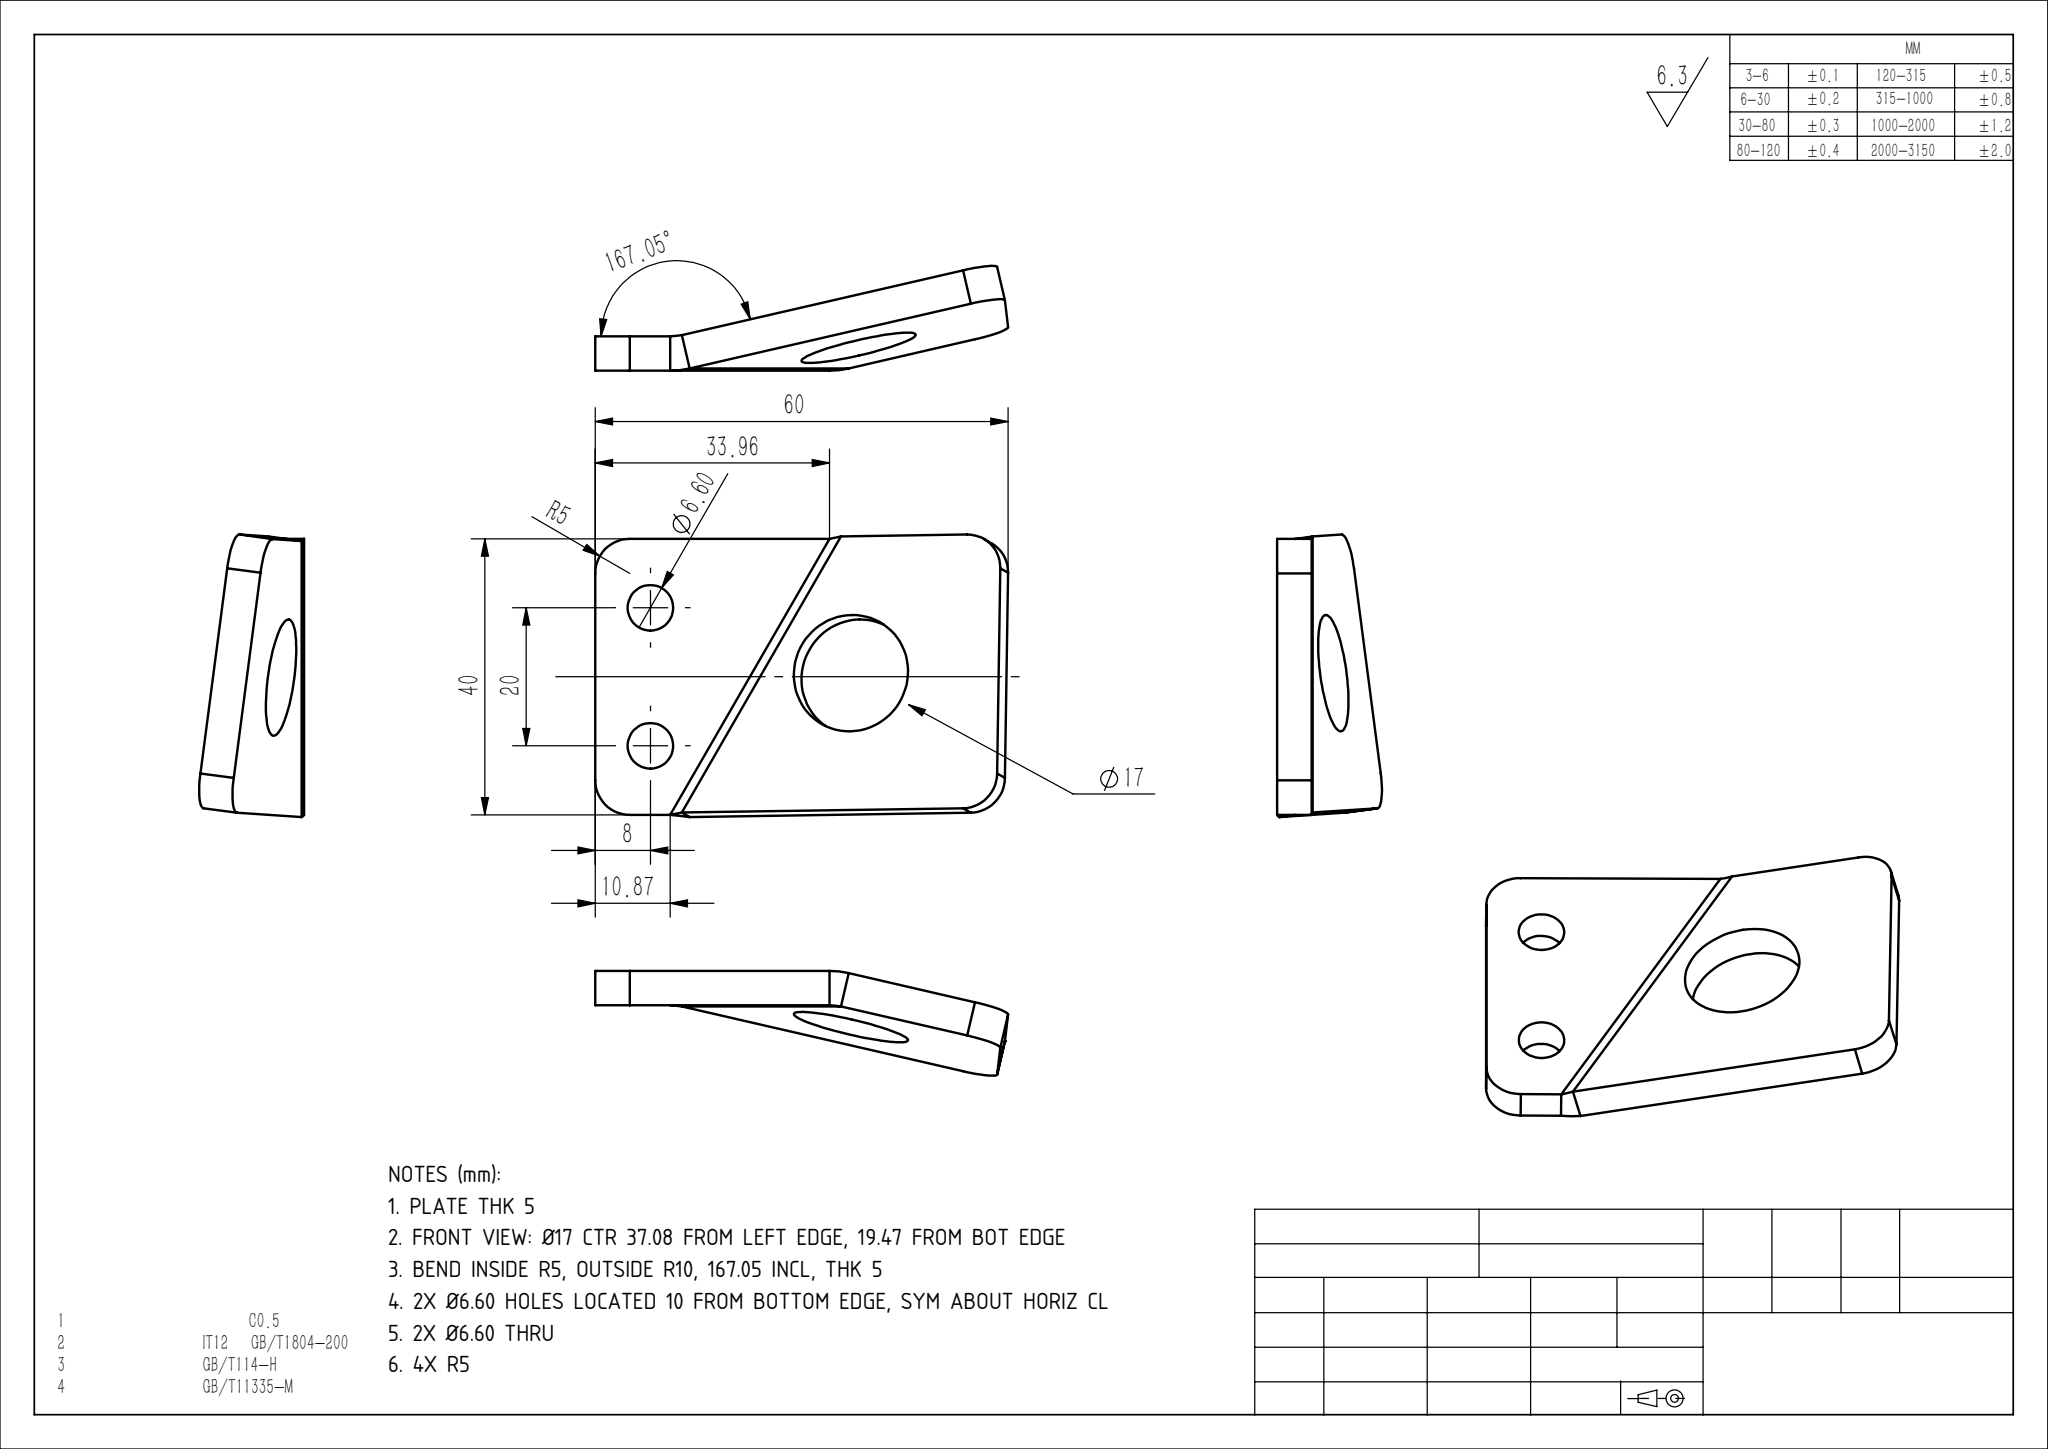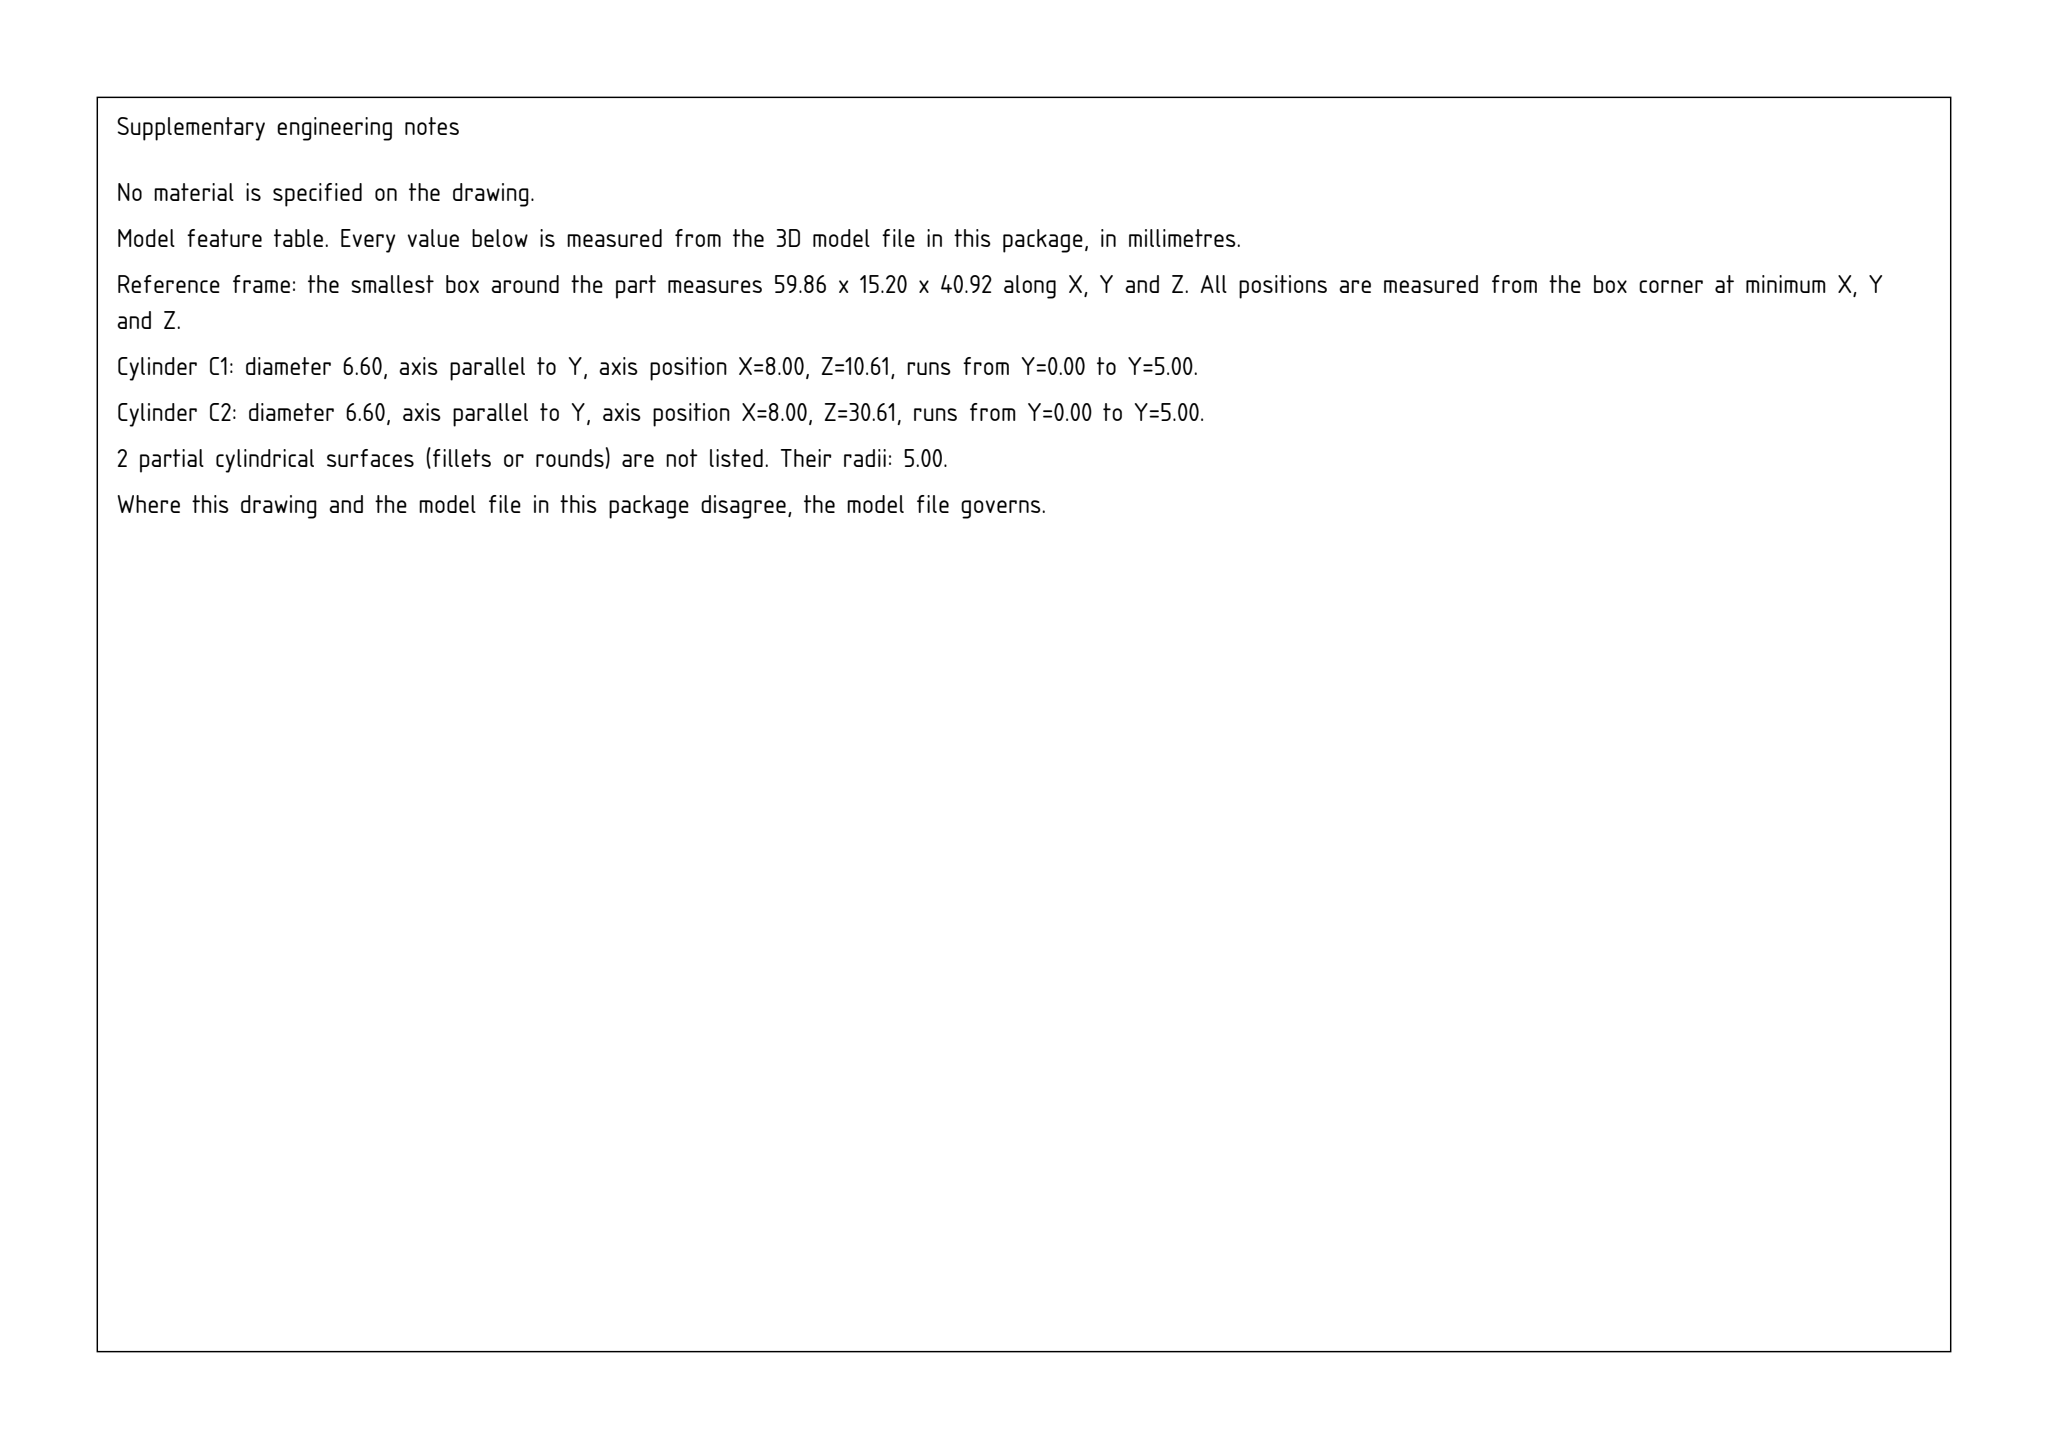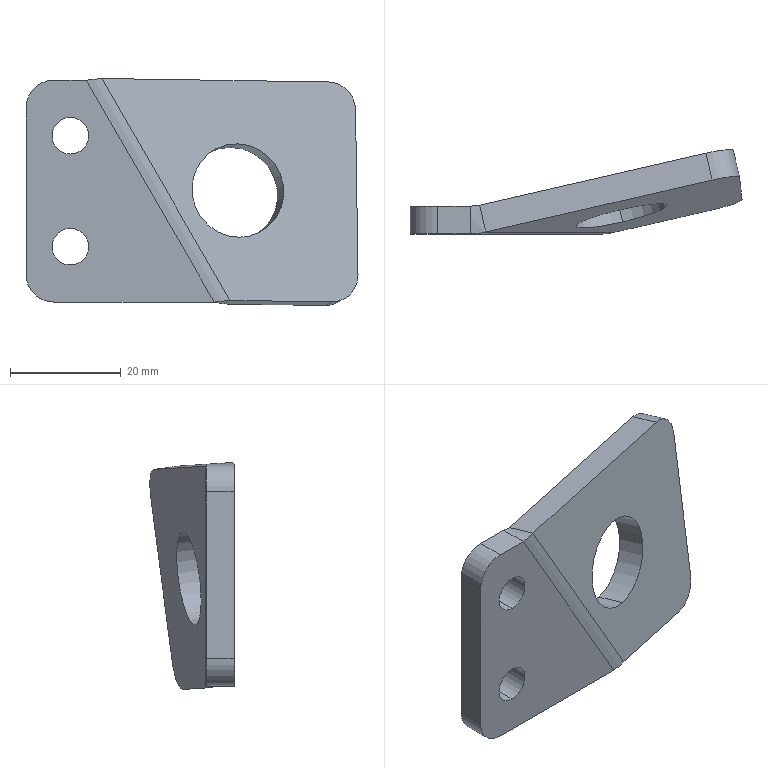Part | SolidWorks | mm | 1 solid | 24 faces | box 59.86 x 15.2 x 40.92 mm | volume 10416 mm3 | cylinder 12 | plane 10 | spline 2 | commonest cylinder face diameters 10 x5 6.6 x4 17 x2 20 x1
Drawing notes:
PLATE THK 5 | from the solid: Parallel faces at y=0 and y=5; all Ø6.60 holes 5 deep
FRONT VIEW: Ø17 CTR 37.08 FROM LEFT EDGE, 19.47 FROM BOT EDGE | from the solid: Ø17 cyl axis Y at x=37.08, z=20.45; part edges at x=0 and z=0.98 (40 wide to z=40.98)
BEND INSIDE R5, OUTSIDE R10, 167.05 INCL, THK 5 | from the solid: Coaxial cyls Ø10 (L=41.63) and Ø20 (L=42.28) about same axis at y=10, x=-1.4; faces y=0/y=5
2X Ø6.60 HOLES LOCATED 10 FROM BOTTOM EDGE, SYM ABOUT HORIZ CL | from the solid: Ø6.6 y-axis cyls at z=10.98 & 30.98; faces z=0.98 & 40.98 (40 wide) -> 10 & 30 from bottom edge, CL at 20.98
2X Ø6.60 THRU | from the solid: two Ø6.6 cylinders, axis y, length 5.0 = plate thk (planes y=0 and y=5)
4X R5 | from the solid: four Ø10 y-axis corner cyls at (5,5.98),(5,35.98),(53.42,35.07),(53.87,5.33)
STEP:
#1=CARTESIAN_POINT('',(8.,0.,6.7));
#2=VERTEX_POINT('',#1);
#3=CARTESIAN_POINT('',(8.,0.,13.3));
#4=VERTEX_POINT('',#3);
#5=CARTESIAN_POINT('',(8.,0.,10.));
#6=DIRECTION('',(0.,1.,0.));
#7=DIRECTION('',(0.,0.,1.));
#8=AXIS2_PLACEMENT_3D('',#5,#6,#7);
#9=CIRCLE('',#8,3.3);
#10=EDGE_CURVE('',#2,#4,#9,.T.);
#11=ORIENTED_EDGE('',*,*,#10,.F.);
#12=CARTESIAN_POINT('',(8.,5.,6.7));
#13=VERTEX_POINT('',#12);
#14=CARTESIAN_POINT('',(8.,5.,6.7));
#15=DIRECTION('',(0.,1.,0.));
#16=VECTOR('',#15,1000.);
#17=LINE('',#14,#16);
#18=EDGE_CURVE('',#2,#13,#17,.T.);
#19=ORIENTED_EDGE('',*,*,#18,.T.);
#20=CARTESIAN_POINT('',(8.,5.,13.3));
#21=VERTEX_POINT('',#20);
#22=CARTESIAN_POINT('',(8.,5.,10.));
#23=DIRECTION('',(0.,1.,0.));
#24=DIRECTION('',(0.,0.,1.));
#25=AXIS2_PLACEMENT_3D('',#22,#23,#24);
#26=CIRCLE('',#25,3.3);
#27=EDGE_CURVE('',#13,#21,#26,.T.);
#28=ORIENTED_EDGE('',*,*,#27,.T.);
#29=CARTESIAN_POINT('',(8.,5.,13.3));
#30=DIRECTION('',(0.,1.,0.));
#31=VECTOR('',#30,1000.);
#32=LINE('',#29,#31);
#33=EDGE_CURVE('',#4,#21,#32,.T.);
#34=ORIENTED_EDGE('',*,*,#33,.F.);
#35=EDGE_LOOP('',(#11,#19,#28,#34));
#36=FACE_OUTER_BOUND('',#35,.T.);
#37=CARTESIAN_POINT('',(8.,5.,10.));
#38=DIRECTION('',(0.,1.,0.));
#39=DIRECTION('',(0.,0.,1.));
#40=AXIS2_PLACEMENT_3D('',#37,#38,#39);
#41=CYLINDRICAL_SURFACE('',#40,3.3);
#42=ADVANCED_FACE('',(#36),#41,.F.);
#43=CARTESIAN_POINT('',(8.,0.,26.7));
#44=VERTEX_POINT('',#43);
#45=CARTESIAN_POINT('',(8.,0.,33.3));
#46=VERTEX_POINT('',#45);
#47=CARTESIAN_POINT('',(8.,0.,30.));
#48=DIRECTION('',(0.,1.,0.));
#49=DIRECTION('',(0.,0.,1.));
#50=AXIS2_PLACEMENT_3D('',#47,#48,#49);
#51=CIRCLE('',#50,3.3);
#52=EDGE_CURVE('',#44,#46,#51,.T.);
#53=ORIENTED_EDGE('',*,*,#52,.F.);
#54=CARTESIAN_POINT('',(8.,5.,26.7));
#55=VERTEX_POINT('',#54);
#56=CARTESIAN_POINT('',(8.,5.,26.7));
#57=DIRECTION('',(0.,1.,0.));
#58=VECTOR('',#57,1000.);
#59=LINE('',#56,#58);
#60=EDGE_CURVE('',#44,#55,#59,.T.);
#61=ORIENTED_EDGE('',*,*,#60,.T.);
#62=CARTESIAN_POINT('',(8.,5.,33.3));
#63=VERTEX_POINT('',#62);
#64=CARTESIAN_POINT('',(8.,5.,30.));
#65=DIRECTION('',(0.,1.,0.));
#66=DIRECTION('',(0.,0.,1.));
#67=AXIS2_PLACEMENT_3D('',#64,#65,#66);
#68=CIRCLE('',#67,3.3);
#69=EDGE_CURVE('',#55,#63,#68,.T.);
#70=ORIENTED_EDGE('',*,*,#69,.T.);
#71=CARTESIAN_POINT('',(8.,5.,33.3));
#72=DIRECTION('',(0.,1.,0.));
#73=VECTOR('',#72,1000.);
#74=LINE('',#71,#73);
#75=EDGE_CURVE('',#46,#63,#74,.T.);
#76=ORIENTED_EDGE('',*,*,#75,.F.);
#77=EDGE_LOOP('',(#53,#61,#70,#76));
#78=FACE_OUTER_BOUND('',#77,.T.);
#79=CARTESIAN_POINT('',(8.,5.,30.));
#80=DIRECTION('',(0.,1.,0.));
#81=DIRECTION('',(0.,0.,1.));
#82=AXIS2_PLACEMENT_3D('',#79,#80,#81);
#83=CYLINDRICAL_SURFACE('',#82,3.3);
#84=ADVANCED_FACE('',(#78),#83,.F.);
#85=CARTESIAN_POINT('',(36.954,9.256,27.896));
#86=VERTEX_POINT('',#85);
#87=CARTESIAN_POINT('',(37.205,7.056,11.041));
#88=VERTEX_POINT('',#87);
#89=CARTESIAN_POINT('',(37.08,8.156,19.469));
#90=DIRECTION('',(0.2241,-0.9659,0.1294));
#91=DIRECTION('',(0.01475,-0.1294,-0.9915));
#92=AXIS2_PLACEMENT_3D('',#89,#90,#91);
#93=CIRCLE('',#92,8.5);
#94=EDGE_CURVE('',#86,#88,#93,.T.);
#95=ORIENTED_EDGE('',*,*,#94,.F.);
#96=CARTESIAN_POINT('',(38.075,4.426,28.543));
#97=VERTEX_POINT('',#96);
#98=CARTESIAN_POINT('',(36.954,9.256,27.896));
#99=DIRECTION('',(0.2241,-0.9659,0.1294));
#100=VECTOR('',#99,1000.);
#101=LINE('',#98,#100);
#102=EDGE_CURVE('',#86,#97,#101,.T.);
#103=ORIENTED_EDGE('',*,*,#102,.T.);
#104=CARTESIAN_POINT('',(38.326,2.226,11.688));
#105=VERTEX_POINT('',#104);
#106=CARTESIAN_POINT('',(38.201,3.326,20.116));
#107=DIRECTION('',(0.2241,-0.9659,0.1294));
#108=DIRECTION('',(0.01475,-0.1294,-0.9915));
#109=AXIS2_PLACEMENT_3D('',#106,#107,#108);
#110=CIRCLE('',#109,8.5);
#111=EDGE_CURVE('',#97,#105,#110,.T.);
#112=ORIENTED_EDGE('',*,*,#111,.T.);
#113=CARTESIAN_POINT('',(37.205,7.056,11.041));
#114=DIRECTION('',(0.2241,-0.9659,0.1294));
#115=VECTOR('',#114,1000.);
#116=LINE('',#113,#115);
#117=EDGE_CURVE('',#88,#105,#116,.T.);
#118=ORIENTED_EDGE('',*,*,#117,.F.);
#119=EDGE_LOOP('',(#95,#103,#112,#118));
#120=FACE_OUTER_BOUND('',#119,.T.);
#121=CARTESIAN_POINT('',(37.08,8.156,19.469));
#122=DIRECTION('',(0.2241,-0.9659,0.1294));
#123=DIRECTION('',(0.01475,-0.1294,-0.9915));
#124=AXIS2_PLACEMENT_3D('',#121,#122,#123);
#125=CYLINDRICAL_SURFACE('',#124,8.5);
#126=ADVANCED_FACE('',(#120),#125,.F.);
#127=CARTESIAN_POINT('',(36.769,0.3407,0.3123));
#128=VERTEX_POINT('',#127);
#129=CARTESIAN_POINT('',(55.061,4.548,0.03537));
#130=VERTEX_POINT('',#129);
#131=CARTESIAN_POINT('',(1.467,-7.779,0.8469));
#132=DIRECTION('',(0.9744,0.2241,-0.01475));
#133=VECTOR('',#132,1000.);
#134=LINE('',#131,#133);
#135=EDGE_CURVE('',#128,#130,#134,.T.);
#136=ORIENTED_EDGE('',*,*,#135,.F.);
#137=CARTESIAN_POINT('',(35.648,5.17,-0.3347));
#138=VERTEX_POINT('',#137);
#139=CARTESIAN_POINT('',(36.769,0.3407,0.3123));
#140=CARTESIAN_POINT('',(36.395,1.951,0.09666));
#141=CARTESIAN_POINT('',(36.021,3.56,-0.119));
#142=CARTESIAN_POINT('',(35.648,5.17,-0.3347));
#143=B_SPLINE_CURVE_WITH_KNOTS('',3,(#139,#140,#141,#142),.UNSPECIFIED.,.F.,.F.,(4,4),(0.,1.),.UNSPECIFIED.);
#144=EDGE_CURVE('',#128,#138,#143,.T.);
#145=ORIENTED_EDGE('',*,*,#144,.T.);
#146=CARTESIAN_POINT('',(53.941,9.378,-0.6117));
#147=VERTEX_POINT('',#146);
#148=CARTESIAN_POINT('',(0.3461,-2.95,0.1998));
#149=DIRECTION('',(0.9744,0.2241,-0.01475));
#150=VECTOR('',#149,1000.);
#151=LINE('',#148,#150);
#152=EDGE_CURVE('',#138,#147,#151,.T.);
#153=ORIENTED_EDGE('',*,*,#152,.T.);
#154=CARTESIAN_POINT('',(53.941,9.378,-0.6117));
#155=DIRECTION('',(-0.2241,0.9659,-0.1294));
#156=VECTOR('',#155,1000.);
#157=LINE('',#154,#156);
#158=EDGE_CURVE('',#130,#147,#157,.T.);
#159=ORIENTED_EDGE('',*,*,#158,.F.);
#160=EDGE_LOOP('',(#136,#145,#153,#159));
#161=FACE_OUTER_BOUND('',#160,.T.);
#162=CARTESIAN_POINT('',(0.3461,-2.95,0.1998));
#163=DIRECTION('',(-0.01475,0.1294,0.9915));
#164=DIRECTION('',(0.9744,0.2241,-0.01475));
#165=AXIS2_PLACEMENT_3D('',#162,#163,#164);
#166=PLANE('',#165);
#167=ADVANCED_FACE('',(#161),#166,.F.);
#168=CARTESIAN_POINT('',(12.554,5.17,39.665));
#169=VERTEX_POINT('',#168);
#170=CARTESIAN_POINT('',(53.35,14.554,39.048));
#171=VERTEX_POINT('',#170);
#172=CARTESIAN_POINT('',(-0.2441,2.227,39.859));
#173=DIRECTION('',(0.9744,0.2241,-0.01475));
#174=VECTOR('',#173,1000.);
#175=LINE('',#172,#174);
#176=EDGE_CURVE('',#169,#171,#175,.T.);
#177=ORIENTED_EDGE('',*,*,#176,.F.);
#178=CARTESIAN_POINT('',(13.675,0.3407,40.312));
#179=VERTEX_POINT('',#178);
#180=CARTESIAN_POINT('',(12.554,5.17,39.665));
#181=CARTESIAN_POINT('',(12.927,3.56,39.881));
#182=CARTESIAN_POINT('',(13.301,1.951,40.097));
#183=CARTESIAN_POINT('',(13.675,0.3407,40.312));
#184=B_SPLINE_CURVE_WITH_KNOTS('',3,(#180,#181,#182,#183),.UNSPECIFIED.,.F.,.F.,(4,4),(0.,1.),.UNSPECIFIED.);
#185=EDGE_CURVE('',#169,#179,#184,.T.);
#186=ORIENTED_EDGE('',*,*,#185,.T.);
#187=CARTESIAN_POINT('',(54.471,9.725,39.695));
#188=VERTEX_POINT('',#187);
#189=CARTESIAN_POINT('',(0.8766,-2.603,40.506));
#190=DIRECTION('',(0.9744,0.2241,-0.01475));
#191=VECTOR('',#190,1000.);
#192=LINE('',#189,#191);
#193=EDGE_CURVE('',#179,#188,#192,.T.);
#194=ORIENTED_EDGE('',*,*,#193,.T.);
#195=CARTESIAN_POINT('',(53.35,14.554,39.048));
#196=DIRECTION('',(-0.2241,0.9659,-0.1294));
#197=VECTOR('',#196,1000.);
#198=LINE('',#195,#197);
#199=EDGE_CURVE('',#188,#171,#198,.T.);
#200=ORIENTED_EDGE('',*,*,#199,.T.);
#201=EDGE_LOOP('',(#177,#186,#194,#200));
#202=FACE_OUTER_BOUND('',#201,.T.);
#203=CARTESIAN_POINT('',(-0.2441,2.227,39.859));
#204=DIRECTION('',(-0.01475,0.1294,0.9915));
#205=DIRECTION('',(0.9744,0.2241,-0.01475));
#206=AXIS2_PLACEMENT_3D('',#203,#204,#205);
#207=PLANE('',#206);
#208=ADVANCED_FACE('',(#202),#207,.T.);
#209=CARTESIAN_POINT('',(37.08,8.156,19.469));
#210=DIRECTION('',(0.2241,-0.9659,0.1294));
#211=DIRECTION('',(0.01475,-0.1294,-0.9915));
#212=AXIS2_PLACEMENT_3D('',#209,#210,#211);
#213=CIRCLE('',#212,8.5);
#214=EDGE_CURVE('',#88,#86,#213,.T.);
#215=ORIENTED_EDGE('',*,*,#214,.T.);
#216=ORIENTED_EDGE('',*,*,#94,.T.);
#217=EDGE_LOOP('',(#215,#216));
#218=FACE_BOUND('',#217,.T.);
#219=ORIENTED_EDGE('',*,*,#152,.F.);
#220=CARTESIAN_POINT('',(9.271,5.17,45.352));
#221=DIRECTION('',(-0.5,0.,0.866));
#222=VECTOR('',#221,1000.);
#223=LINE('',#220,#222);
#224=EDGE_CURVE('',#138,#169,#223,.T.);
#225=ORIENTED_EDGE('',*,*,#224,.T.);
#226=ORIENTED_EDGE('',*,*,#176,.T.);
#227=CARTESIAN_POINT('',(58.296,15.028,34.016));
#228=VERTEX_POINT('',#227);
#229=CARTESIAN_POINT('',(53.424,13.907,34.09));
#230=DIRECTION('',(-0.2241,0.9659,-0.1294));
#231=DIRECTION('',(-0.01475,0.1294,0.9915));
#232=AXIS2_PLACEMENT_3D('',#229,#230,#231);
#233=CIRCLE('',#232,5.);
#234=EDGE_CURVE('',#171,#228,#233,.T.);
#235=ORIENTED_EDGE('',*,*,#234,.T.);
#236=CARTESIAN_POINT('',(58.739,11.146,4.272));
#237=VERTEX_POINT('',#236);
#238=CARTESIAN_POINT('',(58.223,15.675,38.974));
#239=DIRECTION('',(0.01475,-0.1294,-0.9915));
#240=VECTOR('',#239,1000.);
#241=LINE('',#238,#240);
#242=EDGE_CURVE('',#228,#237,#241,.T.);
#243=ORIENTED_EDGE('',*,*,#242,.T.);
#244=CARTESIAN_POINT('',(53.867,10.025,4.346));
#245=DIRECTION('',(-0.2241,0.9659,-0.1294));
#246=DIRECTION('',(-0.01475,0.1294,0.9915));
#247=AXIS2_PLACEMENT_3D('',#244,#245,#246);
#248=CIRCLE('',#247,5.);
#249=EDGE_CURVE('',#237,#147,#248,.T.);
#250=ORIENTED_EDGE('',*,*,#249,.T.);
#251=EDGE_LOOP('',(#219,#225,#226,#235,#243,#250));
#252=FACE_OUTER_BOUND('',#251,.T.);
#253=CARTESIAN_POINT('',(-0.2441,2.227,39.859));
#254=DIRECTION('',(-0.2241,0.9659,-0.1294));
#255=DIRECTION('',(-0.01475,0.1294,0.9915));
#256=AXIS2_PLACEMENT_3D('',#253,#254,#255);
#257=PLANE('',#256);
#258=ADVANCED_FACE('',(#218,#252),#257,.T.);
#259=ORIENTED_EDGE('',*,*,#199,.F.);
#260=CARTESIAN_POINT('',(59.417,10.199,34.663));
#261=VERTEX_POINT('',#260);
#262=CARTESIAN_POINT('',(54.545,9.078,34.737));
#263=DIRECTION('',(-0.2241,0.9659,-0.1294));
#264=DIRECTION('',(-0.01475,0.1294,0.9915));
#265=AXIS2_PLACEMENT_3D('',#262,#263,#264);
#266=CIRCLE('',#265,5.);
#267=EDGE_CURVE('',#188,#261,#266,.T.);
#268=ORIENTED_EDGE('',*,*,#267,.T.);
#269=CARTESIAN_POINT('',(58.296,15.028,34.016));
#270=DIRECTION('',(-0.2241,0.9659,-0.1294));
#271=VECTOR('',#270,1000.);
#272=LINE('',#269,#271);
#273=EDGE_CURVE('',#261,#228,#272,.T.);
#274=ORIENTED_EDGE('',*,*,#273,.T.);
#275=ORIENTED_EDGE('',*,*,#234,.F.);
#276=EDGE_LOOP('',(#259,#268,#274,#275));
#277=FACE_OUTER_BOUND('',#276,.T.);
#278=CARTESIAN_POINT('',(53.424,13.907,34.09));
#279=DIRECTION('',(-0.2241,0.9659,-0.1294));
#280=DIRECTION('',(-0.01475,0.1294,0.9915));
#281=AXIS2_PLACEMENT_3D('',#278,#279,#280);
#282=CYLINDRICAL_SURFACE('',#281,5.);
#283=ADVANCED_FACE('',(#277),#282,.T.);
#284=ORIENTED_EDGE('',*,*,#273,.F.);
#285=CARTESIAN_POINT('',(59.86,6.316,4.919));
#286=VERTEX_POINT('',#285);
#287=CARTESIAN_POINT('',(59.343,10.846,39.621));
#288=DIRECTION('',(0.01475,-0.1294,-0.9915));
#289=VECTOR('',#288,1000.);
#290=LINE('',#287,#289);
#291=EDGE_CURVE('',#261,#286,#290,.T.);
#292=ORIENTED_EDGE('',*,*,#291,.T.);
#293=CARTESIAN_POINT('',(58.739,11.146,4.272));
#294=DIRECTION('',(-0.2241,0.9659,-0.1294));
#295=VECTOR('',#294,1000.);
#296=LINE('',#293,#295);
#297=EDGE_CURVE('',#286,#237,#296,.T.);
#298=ORIENTED_EDGE('',*,*,#297,.T.);
#299=ORIENTED_EDGE('',*,*,#242,.F.);
#300=EDGE_LOOP('',(#284,#292,#298,#299));
#301=FACE_OUTER_BOUND('',#300,.T.);
#302=CARTESIAN_POINT('',(58.223,15.675,38.974));
#303=DIRECTION('',(0.9744,0.2241,-0.01475));
#304=DIRECTION('',(0.01475,-0.1294,-0.9915));
#305=AXIS2_PLACEMENT_3D('',#302,#303,#304);
#306=PLANE('',#305);
#307=ADVANCED_FACE('',(#301),#306,.T.);
#308=ORIENTED_EDGE('',*,*,#102,.F.);
#309=ORIENTED_EDGE('',*,*,#214,.F.);
#310=ORIENTED_EDGE('',*,*,#117,.T.);
#311=CARTESIAN_POINT('',(38.201,3.326,20.116));
#312=DIRECTION('',(0.2241,-0.9659,0.1294));
#313=DIRECTION('',(0.01475,-0.1294,-0.9915));
#314=AXIS2_PLACEMENT_3D('',#311,#312,#313);
#315=CIRCLE('',#314,8.5);
#316=EDGE_CURVE('',#105,#97,#315,.T.);
#317=ORIENTED_EDGE('',*,*,#316,.T.);
#318=EDGE_LOOP('',(#308,#309,#310,#317));
#319=FACE_OUTER_BOUND('',#318,.T.);
#320=CARTESIAN_POINT('',(37.08,8.156,19.469));
#321=DIRECTION('',(0.2241,-0.9659,0.1294));
#322=DIRECTION('',(0.01475,-0.1294,-0.9915));
#323=AXIS2_PLACEMENT_3D('',#320,#321,#322);
#324=CYLINDRICAL_SURFACE('',#323,8.5);
#325=ADVANCED_FACE('',(#319),#324,.F.);
#326=CARTESIAN_POINT('',(54.987,5.195,4.993));
#327=DIRECTION('',(-0.2241,0.9659,-0.1294));
#328=DIRECTION('',(-0.01475,0.1294,0.9915));
#329=AXIS2_PLACEMENT_3D('',#326,#327,#328);
#330=CIRCLE('',#329,5.);
#331=EDGE_CURVE('',#286,#130,#330,.T.);
#332=ORIENTED_EDGE('',*,*,#331,.T.);
#333=ORIENTED_EDGE('',*,*,#158,.T.);
#334=ORIENTED_EDGE('',*,*,#249,.F.);
#335=ORIENTED_EDGE('',*,*,#297,.F.);
#336=EDGE_LOOP('',(#332,#333,#334,#335));
#337=FACE_OUTER_BOUND('',#336,.T.);
#338=CARTESIAN_POINT('',(53.867,10.025,4.346));
#339=DIRECTION('',(-0.2241,0.9659,-0.1294));
#340=DIRECTION('',(-0.01475,0.1294,0.9915));
#341=AXIS2_PLACEMENT_3D('',#338,#339,#340);
#342=CYLINDRICAL_SURFACE('',#341,5.);
#343=ADVANCED_FACE('',(#337),#342,.T.);
#344=CARTESIAN_POINT('',(10.391,0.3407,45.999));
#345=DIRECTION('',(-0.5,0.,0.866));
#346=VECTOR('',#345,1000.);
#347=LINE('',#344,#346);
#348=EDGE_CURVE('',#128,#179,#347,.T.);
#349=ORIENTED_EDGE('',*,*,#348,.F.);
#350=ORIENTED_EDGE('',*,*,#135,.T.);
#351=ORIENTED_EDGE('',*,*,#331,.F.);
#352=ORIENTED_EDGE('',*,*,#291,.F.);
#353=ORIENTED_EDGE('',*,*,#267,.F.);
#354=ORIENTED_EDGE('',*,*,#193,.F.);
#355=EDGE_LOOP('',(#349,#350,#351,#352,#353,#354));
#356=FACE_OUTER_BOUND('',#355,.T.);
#357=ORIENTED_EDGE('',*,*,#316,.F.);
#358=ORIENTED_EDGE('',*,*,#111,.F.);
#359=EDGE_LOOP('',(#357,#358));
#360=FACE_BOUND('',#359,.T.);
#361=CARTESIAN_POINT('',(0.8766,-2.603,40.506));
#362=DIRECTION('',(-0.2241,0.9659,-0.1294));
#363=DIRECTION('',(-0.01475,0.1294,0.9915));
#364=AXIS2_PLACEMENT_3D('',#361,#362,#363);
#365=PLANE('',#364);
#366=ADVANCED_FACE('',(#356,#360),#365,.F.);
#367=ORIENTED_EDGE('',*,*,#60,.F.);
#368=CARTESIAN_POINT('',(8.,0.,30.));
#369=DIRECTION('',(0.,1.,0.));
#370=DIRECTION('',(0.,0.,1.));
#371=AXIS2_PLACEMENT_3D('',#368,#369,#370);
#372=CIRCLE('',#371,3.3);
#373=EDGE_CURVE('',#46,#44,#372,.T.);
#374=ORIENTED_EDGE('',*,*,#373,.F.);
#375=ORIENTED_EDGE('',*,*,#75,.T.);
#376=CARTESIAN_POINT('',(8.,5.,30.));
#377=DIRECTION('',(0.,1.,0.));
#378=DIRECTION('',(0.,0.,1.));
#379=AXIS2_PLACEMENT_3D('',#376,#377,#378);
#380=CIRCLE('',#379,3.3);
#381=EDGE_CURVE('',#63,#55,#380,.T.);
#382=ORIENTED_EDGE('',*,*,#381,.T.);
#383=EDGE_LOOP('',(#367,#374,#375,#382));
#384=FACE_OUTER_BOUND('',#383,.T.);
#385=CARTESIAN_POINT('',(8.,5.,30.));
#386=DIRECTION('',(0.,1.,0.));
#387=DIRECTION('',(0.,0.,1.));
#388=AXIS2_PLACEMENT_3D('',#385,#386,#387);
#389=CYLINDRICAL_SURFACE('',#388,3.3);
#390=ADVANCED_FACE('',(#384),#389,.F.);
#391=ORIENTED_EDGE('',*,*,#18,.F.);
#392=CARTESIAN_POINT('',(8.,0.,10.));
#393=DIRECTION('',(0.,1.,0.));
#394=DIRECTION('',(0.,0.,1.));
#395=AXIS2_PLACEMENT_3D('',#392,#393,#394);
#396=CIRCLE('',#395,3.3);
#397=EDGE_CURVE('',#4,#2,#396,.T.);
#398=ORIENTED_EDGE('',*,*,#397,.F.);
#399=ORIENTED_EDGE('',*,*,#33,.T.);
#400=CARTESIAN_POINT('',(8.,5.,10.));
#401=DIRECTION('',(0.,1.,0.));
#402=DIRECTION('',(0.,0.,1.));
#403=AXIS2_PLACEMENT_3D('',#400,#401,#402);
#404=CIRCLE('',#403,3.3);
#405=EDGE_CURVE('',#21,#13,#404,.T.);
#406=ORIENTED_EDGE('',*,*,#405,.T.);
#407=EDGE_LOOP('',(#391,#398,#399,#406));
#408=FACE_OUTER_BOUND('',#407,.T.);
#409=CARTESIAN_POINT('',(8.,5.,10.));
#410=DIRECTION('',(0.,1.,0.));
#411=DIRECTION('',(0.,0.,1.));
#412=AXIS2_PLACEMENT_3D('',#409,#410,#411);
#413=CYLINDRICAL_SURFACE('',#412,3.3);
#414=ADVANCED_FACE('',(#408),#413,.F.);
#415=CARTESIAN_POINT('',(0.,0.,35.));
#416=VERTEX_POINT('',#415);
#417=CARTESIAN_POINT('',(0.,5.,35.));
#418=VERTEX_POINT('',#417);
#419=CARTESIAN_POINT('',(0.,5.,35.));
#420=DIRECTION('',(0.,1.,0.));
#421=VECTOR('',#420,1000.);
#422=LINE('',#419,#421);
#423=EDGE_CURVE('',#416,#418,#422,.T.);
#424=ORIENTED_EDGE('',*,*,#423,.F.);
#425=CARTESIAN_POINT('',(5.,0.,40.));
#426=VERTEX_POINT('',#425);
#427=CARTESIAN_POINT('',(5.,0.,35.));
#428=DIRECTION('',(0.,1.,0.));
#429=DIRECTION('',(0.,0.,1.));
#430=AXIS2_PLACEMENT_3D('',#427,#428,#429);
#431=CIRCLE('',#430,5.);
#432=EDGE_CURVE('',#416,#426,#431,.T.);
#433=ORIENTED_EDGE('',*,*,#432,.T.);
#434=CARTESIAN_POINT('',(5.,5.,40.));
#435=VERTEX_POINT('',#434);
#436=CARTESIAN_POINT('',(5.,5.,40.));
#437=DIRECTION('',(0.,1.,0.));
#438=VECTOR('',#437,1000.);
#439=LINE('',#436,#438);
#440=EDGE_CURVE('',#426,#435,#439,.T.);
#441=ORIENTED_EDGE('',*,*,#440,.T.);
#442=CARTESIAN_POINT('',(5.,5.,35.));
#443=DIRECTION('',(0.,1.,0.));
#444=DIRECTION('',(0.,0.,1.));
#445=AXIS2_PLACEMENT_3D('',#442,#443,#444);
#446=CIRCLE('',#445,5.);
#447=EDGE_CURVE('',#418,#435,#446,.T.);
#448=ORIENTED_EDGE('',*,*,#447,.F.);
#449=EDGE_LOOP('',(#424,#433,#441,#448));
#450=FACE_OUTER_BOUND('',#449,.T.);
#451=CARTESIAN_POINT('',(5.,5.,35.));
#452=DIRECTION('',(0.,1.,0.));
#453=DIRECTION('',(0.,0.,1.));
#454=AXIS2_PLACEMENT_3D('',#451,#452,#453);
#455=CYLINDRICAL_SURFACE('',#454,5.);
#456=ADVANCED_FACE('',(#450),#455,.T.);
#457=CARTESIAN_POINT('',(0.,0.,5.));
#458=VERTEX_POINT('',#457);
#459=CARTESIAN_POINT('',(0.,5.,5.));
#460=VERTEX_POINT('',#459);
#461=CARTESIAN_POINT('',(0.,5.,5.));
#462=DIRECTION('',(0.,1.,0.));
#463=VECTOR('',#462,1000.);
#464=LINE('',#461,#463);
#465=EDGE_CURVE('',#458,#460,#464,.T.);
#466=ORIENTED_EDGE('',*,*,#465,.F.);
#467=CARTESIAN_POINT('',(0.,0.,40.));
#468=DIRECTION('',(0.,0.,-1.));
#469=VECTOR('',#468,1000.);
#470=LINE('',#467,#469);
#471=EDGE_CURVE('',#416,#458,#470,.T.);
#472=ORIENTED_EDGE('',*,*,#471,.F.);
#473=ORIENTED_EDGE('',*,*,#423,.T.);
#474=CARTESIAN_POINT('',(0.,5.,40.));
#475=DIRECTION('',(0.,0.,-1.));
#476=VECTOR('',#475,1000.);
#477=LINE('',#474,#476);
#478=EDGE_CURVE('',#418,#460,#477,.T.);
#479=ORIENTED_EDGE('',*,*,#478,.T.);
#480=EDGE_LOOP('',(#466,#472,#473,#479));
#481=FACE_OUTER_BOUND('',#480,.T.);
#482=CARTESIAN_POINT('',(0.,5.,40.));
#483=DIRECTION('',(1.,0.,0.));
#484=DIRECTION('',(0.,0.,-1.));
#485=AXIS2_PLACEMENT_3D('',#482,#483,#484);
#486=PLANE('',#485);
#487=ADVANCED_FACE('',(#481),#486,.F.);
#488=CARTESIAN_POINT('',(5.,0.,0.));
#489=VERTEX_POINT('',#488);
#490=CARTESIAN_POINT('',(5.,5.,0.));
#491=VERTEX_POINT('',#490);
#492=CARTESIAN_POINT('',(5.,5.,0.));
#493=DIRECTION('',(0.,1.,0.));
#494=VECTOR('',#493,1000.);
#495=LINE('',#492,#494);
#496=EDGE_CURVE('',#489,#491,#495,.T.);
#497=ORIENTED_EDGE('',*,*,#496,.F.);
#498=CARTESIAN_POINT('',(5.,0.,5.));
#499=DIRECTION('',(0.,1.,0.));
#500=DIRECTION('',(0.,0.,1.));
#501=AXIS2_PLACEMENT_3D('',#498,#499,#500);
#502=CIRCLE('',#501,5.);
#503=EDGE_CURVE('',#489,#458,#502,.T.);
#504=ORIENTED_EDGE('',*,*,#503,.T.);
#505=ORIENTED_EDGE('',*,*,#465,.T.);
#506=CARTESIAN_POINT('',(5.,5.,5.));
#507=DIRECTION('',(0.,1.,0.));
#508=DIRECTION('',(0.,0.,1.));
#509=AXIS2_PLACEMENT_3D('',#506,#507,#508);
#510=CIRCLE('',#509,5.);
#511=EDGE_CURVE('',#491,#460,#510,.T.);
#512=ORIENTED_EDGE('',*,*,#511,.F.);
#513=EDGE_LOOP('',(#497,#504,#505,#512));
#514=FACE_OUTER_BOUND('',#513,.T.);
#515=CARTESIAN_POINT('',(5.,5.,5.));
#516=DIRECTION('',(0.,1.,0.));
#517=DIRECTION('',(0.,0.,1.));
#518=AXIS2_PLACEMENT_3D('',#515,#516,#517);
#519=CYLINDRICAL_SURFACE('',#518,5.);
#520=ADVANCED_FACE('',(#514),#519,.T.);
#521=CARTESIAN_POINT('',(33.96,5.,-0.));
#522=VERTEX_POINT('',#521);
#523=CARTESIAN_POINT('',(10.866,5.,40.));
#524=VERTEX_POINT('',#523);
#525=CARTESIAN_POINT('',(8.15,5.,44.705));
#526=DIRECTION('',(-0.5,0.,0.866));
#527=VECTOR('',#526,1000.);
#528=LINE('',#525,#527);
#529=EDGE_CURVE('',#522,#524,#528,.T.);
#530=ORIENTED_EDGE('',*,*,#529,.F.);
#531=CARTESIAN_POINT('',(0.,5.,0.));
#532=DIRECTION('',(1.,0.,0.));
#533=VECTOR('',#532,1000.);
#534=LINE('',#531,#533);
#535=EDGE_CURVE('',#491,#522,#534,.T.);
#536=ORIENTED_EDGE('',*,*,#535,.F.);
#537=ORIENTED_EDGE('',*,*,#511,.T.);
#538=ORIENTED_EDGE('',*,*,#478,.F.);
#539=ORIENTED_EDGE('',*,*,#447,.T.);
#540=CARTESIAN_POINT('',(0.,5.,40.));
#541=DIRECTION('',(1.,0.,0.));
#542=VECTOR('',#541,1000.);
#543=LINE('',#540,#542);
#544=EDGE_CURVE('',#435,#524,#543,.T.);
#545=ORIENTED_EDGE('',*,*,#544,.T.);
#546=EDGE_LOOP('',(#530,#536,#537,#538,#539,#545));
#547=FACE_OUTER_BOUND('',#546,.T.);
#548=ORIENTED_EDGE('',*,*,#405,.F.);
#549=ORIENTED_EDGE('',*,*,#27,.F.);
#550=EDGE_LOOP('',(#548,#549));
#551=FACE_BOUND('',#550,.T.);
#552=ORIENTED_EDGE('',*,*,#381,.F.);
#553=ORIENTED_EDGE('',*,*,#69,.F.);
#554=EDGE_LOOP('',(#552,#553));
#555=FACE_BOUND('',#554,.T.);
#556=CARTESIAN_POINT('',(0.,5.,40.));
#557=DIRECTION('',(0.,1.,0.));
#558=DIRECTION('',(0.,0.,1.));
#559=AXIS2_PLACEMENT_3D('',#556,#557,#558);
#560=PLANE('',#559);
#561=ADVANCED_FACE('',(#547,#551,#555),#560,.T.);
#562=CARTESIAN_POINT('',(33.96,0.,-0.));
#563=VERTEX_POINT('',#562);
#564=CARTESIAN_POINT('',(33.96,0.,-0.));
#565=CARTESIAN_POINT('',(33.96,5.,-0.));
#566=B_SPLINE_CURVE_WITH_KNOTS('',1,(#564,#565),.UNSPECIFIED.,.F.,.F.,(2,2),(0.,1.),.UNSPECIFIED.);
#567=EDGE_CURVE('',#563,#522,#566,.T.);
#568=ORIENTED_EDGE('',*,*,#567,.F.);
#569=CARTESIAN_POINT('',(0.,0.,0.));
#570=DIRECTION('',(1.,0.,0.));
#571=VECTOR('',#570,1000.);
#572=LINE('',#569,#571);
#573=EDGE_CURVE('',#489,#563,#572,.T.);
#574=ORIENTED_EDGE('',*,*,#573,.F.);
#575=ORIENTED_EDGE('',*,*,#496,.T.);
#576=ORIENTED_EDGE('',*,*,#535,.T.);
#577=EDGE_LOOP('',(#568,#574,#575,#576));
#578=FACE_OUTER_BOUND('',#577,.T.);
#579=CARTESIAN_POINT('',(0.,5.,0.));
#580=DIRECTION('',(0.,0.,1.));
#581=DIRECTION('',(1.,0.,0.));
#582=AXIS2_PLACEMENT_3D('',#579,#580,#581);
#583=PLANE('',#582);
#584=ADVANCED_FACE('',(#578),#583,.F.);
#585=ORIENTED_EDGE('',*,*,#373,.T.);
#586=ORIENTED_EDGE('',*,*,#52,.T.);
#587=EDGE_LOOP('',(#585,#586));
#588=FACE_BOUND('',#587,.T.);
#589=ORIENTED_EDGE('',*,*,#397,.T.);
#590=ORIENTED_EDGE('',*,*,#10,.T.);
#591=EDGE_LOOP('',(#589,#590));
#592=FACE_BOUND('',#591,.T.);
#593=ORIENTED_EDGE('',*,*,#573,.T.);
#594=CARTESIAN_POINT('',(10.866,0.,40.));
#595=VERTEX_POINT('',#594);
#596=CARTESIAN_POINT('',(8.15,0.,44.705));
#597=DIRECTION('',(-0.5,0.,0.866));
#598=VECTOR('',#597,1000.);
#599=LINE('',#596,#598);
#600=EDGE_CURVE('',#563,#595,#599,.T.);
#601=ORIENTED_EDGE('',*,*,#600,.T.);
#602=CARTESIAN_POINT('',(0.,0.,40.));
#603=DIRECTION('',(1.,0.,0.));
#604=VECTOR('',#603,1000.);
#605=LINE('',#602,#604);
#606=EDGE_CURVE('',#426,#595,#605,.T.);
#607=ORIENTED_EDGE('',*,*,#606,.F.);
#608=ORIENTED_EDGE('',*,*,#432,.F.);
#609=ORIENTED_EDGE('',*,*,#471,.T.);
#610=ORIENTED_EDGE('',*,*,#503,.F.);
#611=EDGE_LOOP('',(#593,#601,#607,#608,#609,#610));
#612=FACE_OUTER_BOUND('',#611,.T.);
#613=CARTESIAN_POINT('',(0.,0.,40.));
#614=DIRECTION('',(0.,1.,0.));
#615=DIRECTION('',(0.,0.,1.));
#616=AXIS2_PLACEMENT_3D('',#613,#614,#615);
#617=PLANE('',#616);
#618=ADVANCED_FACE('',(#588,#592,#612),#617,.F.);
#619=CARTESIAN_POINT('',(10.866,5.,40.));
#620=CARTESIAN_POINT('',(10.866,0.,40.));
#621=B_SPLINE_CURVE_WITH_KNOTS('',1,(#619,#620),.UNSPECIFIED.,.F.,.F.,(2,2),(0.,1.),.UNSPECIFIED.);
#622=EDGE_CURVE('',#524,#595,#621,.T.);
#623=ORIENTED_EDGE('',*,*,#622,.F.);
#624=ORIENTED_EDGE('',*,*,#544,.F.);
#625=ORIENTED_EDGE('',*,*,#440,.F.);
#626=ORIENTED_EDGE('',*,*,#606,.T.);
#627=EDGE_LOOP('',(#623,#624,#625,#626));
#628=FACE_OUTER_BOUND('',#627,.T.);
#629=CARTESIAN_POINT('',(0.,5.,40.));
#630=DIRECTION('',(0.,0.,1.));
#631=DIRECTION('',(1.,0.,0.));
#632=AXIS2_PLACEMENT_3D('',#629,#630,#631);
#633=PLANE('',#632);
#634=ADVANCED_FACE('',(#628),#633,.T.);
#635=ORIENTED_EDGE('',*,*,#144,.F.);
#636=CARTESIAN_POINT('',(36.769,0.3407,0.3123));
#637=CARTESIAN_POINT('',(35.85,0.1149,0.2181));
#638=CARTESIAN_POINT('',(34.905,-0.,0.1091));
#639=CARTESIAN_POINT('',(33.96,0.,-0.));
#640=B_SPLINE_CURVE_WITH_KNOTS('',3,(#636,#637,#638,#639),.UNSPECIFIED.,.F.,.F.,(4,4),(0.,1.),.UNSPECIFIED.);
#641=EDGE_CURVE('',#128,#563,#640,.T.);
#642=ORIENTED_EDGE('',*,*,#641,.T.);
#643=ORIENTED_EDGE('',*,*,#567,.T.);
#644=CARTESIAN_POINT('',(35.648,5.17,-0.3347));
#645=CARTESIAN_POINT('',(35.094,5.057,-0.2182));
#646=CARTESIAN_POINT('',(34.527,5.,-0.1091));
#647=CARTESIAN_POINT('',(33.96,5.,-0.));
#648=B_SPLINE_CURVE_WITH_KNOTS('',3,(#644,#645,#646,#647),.UNSPECIFIED.,.F.,.F.,(4,4),(0.,1.),.UNSPECIFIED.);
#649=EDGE_CURVE('',#138,#522,#648,.T.);
#650=ORIENTED_EDGE('',*,*,#649,.F.);
#651=EDGE_LOOP('',(#635,#642,#643,#650));
#652=FACE_OUTER_BOUND('',#651,.T.);
#653=CARTESIAN_POINT('',(36.769,0.3407,0.3123));
#654=CARTESIAN_POINT('',(35.85,0.1149,0.2181));
#655=CARTESIAN_POINT('',(34.905,-0.,0.1091));
#656=CARTESIAN_POINT('',(33.96,-0.,-0.));
#657=CARTESIAN_POINT('',(35.648,5.17,-0.3347));
#658=CARTESIAN_POINT('',(35.094,5.057,-0.2182));
#659=CARTESIAN_POINT('',(34.527,5.,-0.1091));
#660=CARTESIAN_POINT('',(33.96,5.,-0.));
#661=B_SPLINE_SURFACE_WITH_KNOTS('',1,3,((#653,#654,#655,#656),(#657,#658,#659,#660)),.UNSPECIFIED.,.F.,.F.,.F.,(2,2),(4,4),(0.,1.),(0.,1.),.UNSPECIFIED.);
#662=ADVANCED_FACE('',(#652),#661,.F.);
#663=CARTESIAN_POINT('',(10.866,0.,40.));
#664=CARTESIAN_POINT('',(11.811,-0.,40.109));
#665=CARTESIAN_POINT('',(12.756,0.1149,40.218));
#666=CARTESIAN_POINT('',(13.675,0.3407,40.312));
#667=B_SPLINE_CURVE_WITH_KNOTS('',3,(#663,#664,#665,#666),.UNSPECIFIED.,.F.,.F.,(4,4),(0.,1.),.UNSPECIFIED.);
#668=EDGE_CURVE('',#595,#179,#667,.T.);
#669=ORIENTED_EDGE('',*,*,#668,.T.);
#670=ORIENTED_EDGE('',*,*,#185,.F.);
#671=CARTESIAN_POINT('',(10.866,5.,40.));
#672=CARTESIAN_POINT('',(11.433,5.,39.891));
#673=CARTESIAN_POINT('',(12.,5.057,39.782));
#674=CARTESIAN_POINT('',(12.554,5.17,39.665));
#675=B_SPLINE_CURVE_WITH_KNOTS('',3,(#671,#672,#673,#674),.UNSPECIFIED.,.F.,.F.,(4,4),(0.,1.),.UNSPECIFIED.);
#676=EDGE_CURVE('',#524,#169,#675,.T.);
#677=ORIENTED_EDGE('',*,*,#676,.F.);
#678=ORIENTED_EDGE('',*,*,#622,.T.);
#679=EDGE_LOOP('',(#669,#670,#677,#678));
#680=FACE_OUTER_BOUND('',#679,.T.);
#681=CARTESIAN_POINT('',(10.866,-0.,40.));
#682=CARTESIAN_POINT('',(11.811,-0.,40.109));
#683=CARTESIAN_POINT('',(12.756,0.1149,40.218));
#684=CARTESIAN_POINT('',(13.675,0.3407,40.312));
#685=CARTESIAN_POINT('',(10.866,5.,40.));
#686=CARTESIAN_POINT('',(11.433,5.,39.891));
#687=CARTESIAN_POINT('',(12.,5.057,39.782));
#688=CARTESIAN_POINT('',(12.554,5.17,39.665));
#689=B_SPLINE_SURFACE_WITH_KNOTS('',1,3,((#681,#682,#683,#684),(#685,#686,#687,#688)),.UNSPECIFIED.,.F.,.F.,.F.,(2,2),(4,4),(0.,1.),(0.,1.),.UNSPECIFIED.);
#690=ADVANCED_FACE('',(#680),#689,.F.);
#691=ORIENTED_EDGE('',*,*,#529,.T.);
#692=ORIENTED_EDGE('',*,*,#676,.T.);
#693=ORIENTED_EDGE('',*,*,#224,.F.);
#694=ORIENTED_EDGE('',*,*,#649,.T.);
#695=EDGE_LOOP('',(#691,#692,#693,#694));
#696=FACE_OUTER_BOUND('',#695,.T.);
#697=CARTESIAN_POINT('',(-1.399,10.,61.245));
#698=DIRECTION('',(0.5,0.,-0.866));
#699=DIRECTION('',(-0.866,0.,-0.5));
#700=AXIS2_PLACEMENT_3D('',#697,#698,#699);
#701=CYLINDRICAL_SURFACE('',#700,5.);
#702=ADVANCED_FACE('',(#696),#701,.F.);
#703=ORIENTED_EDGE('',*,*,#600,.F.);
#704=ORIENTED_EDGE('',*,*,#641,.F.);
#705=ORIENTED_EDGE('',*,*,#348,.T.);
#706=ORIENTED_EDGE('',*,*,#668,.F.);
#707=EDGE_LOOP('',(#703,#704,#705,#706));
#708=FACE_OUTER_BOUND('',#707,.T.);
#709=CARTESIAN_POINT('',(-1.399,10.,61.245));
#710=DIRECTION('',(0.5,0.,-0.866));
#711=DIRECTION('',(-0.866,0.,-0.5));
#712=AXIS2_PLACEMENT_3D('',#709,#710,#711);
#713=CYLINDRICAL_SURFACE('',#712,10.);
#714=ADVANCED_FACE('',(#708),#713,.T.);
#715=CLOSED_SHELL('',(#42,#84,#126,#167,#208,#258,#283,#307,#325,#343,#366,#390,#414,#456,#487,#520,#561,#584,#618,#634,#662,#690,#702,#714));
#716=MANIFOLD_SOLID_BREP('',#715);
#717=CARTESIAN_POINT('',(0.,0.,0.));
#718=DIRECTION('',(0.,0.,1.));
#719=DIRECTION('',(1.,0.,0.));
#720=AXIS2_PLACEMENT_3D('',#717,#718,#719);
#721=(LENGTH_UNIT()NAMED_UNIT(*)SI_UNIT(.MILLI.,.METRE.));
#722=UNCERTAINTY_MEASURE_WITH_UNIT(LENGTH_MEASURE(0.00001),#721,'','');
#723=(NAMED_UNIT(*)PLANE_ANGLE_UNIT()SI_UNIT($,.RADIAN.));
#724=(NAMED_UNIT(*)SI_UNIT($,.STERADIAN.)SOLID_ANGLE_UNIT());
#725=(GEOMETRIC_REPRESENTATION_CONTEXT(3)GLOBAL_UNCERTAINTY_ASSIGNED_CONTEXT((#722))GLOBAL_UNIT_ASSIGNED_CONTEXT((#721,#723,#724))REPRESENTATION_CONTEXT('',''));
#726=ADVANCED_BREP_SHAPE_REPRESENTATION('',(#716,#720),#725);